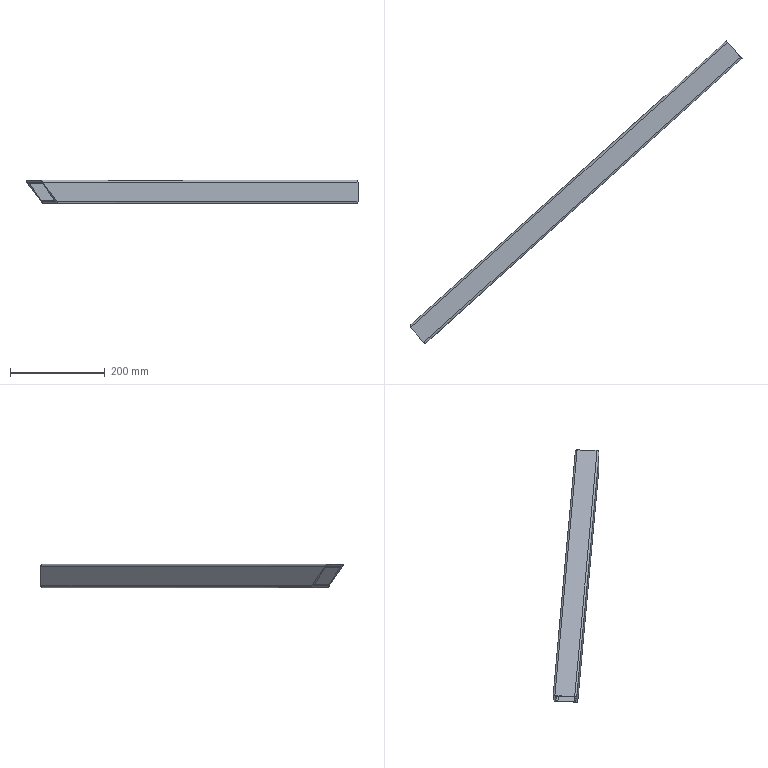Component | NX | ADJ_BRKT_VERT_BEAM | 1 solid | 18 faces | volume 644000 mm3 | plane 10 | cylinder 8 | commonest cylinder face diameters 8 x8